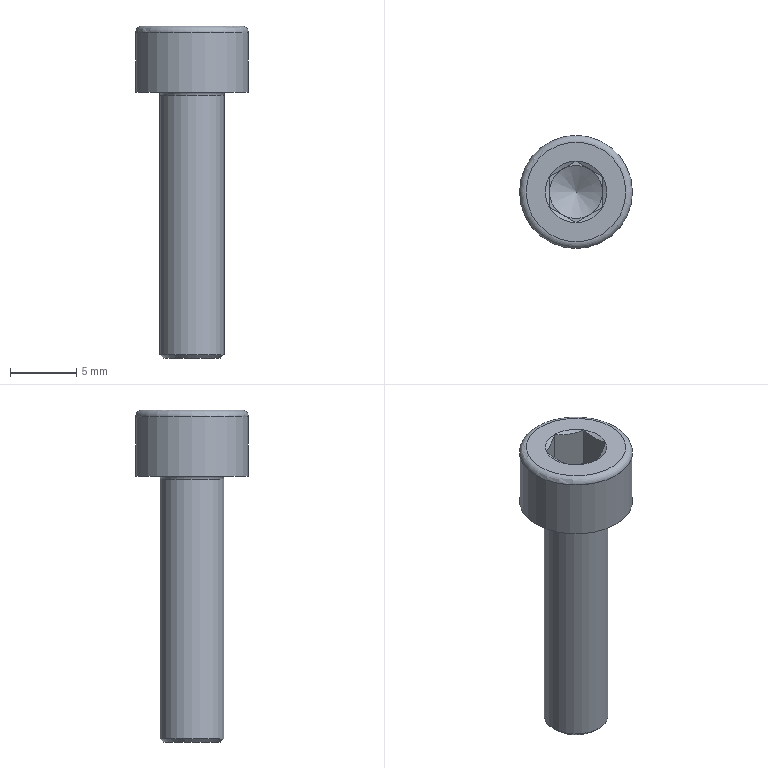Component | NX | GB-T70_1-2000_M5X20 | 1 solid | 27 faces | volume 600 mm3 | plane 15 | cone 8 | cylinder 2 | torus 2 | commonest cylinder face diameters 4.826 x1 8.5 x1